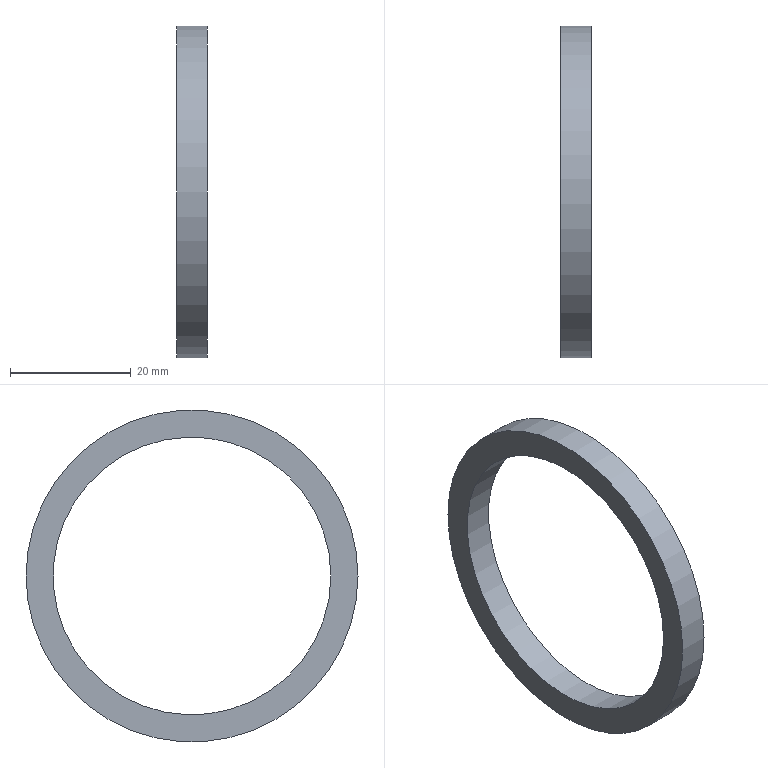Component | NX | XIAOTIAOZHENGHUAN_3 | 1 solid | 4 faces | box 5 x 55 x 55 mm | volume 3570 mm3 | cylinder 2 | plane 2 | commonest cylinder face diameters 55 x1 46 x1
STEP:
#1=CARTESIAN_POINT('',(0.,0.,0.));
#2=DIRECTION('',(0.,0.,1.));
#3=DIRECTION('',(1.,0.,0.));
#4=AXIS2_PLACEMENT_3D('',#1,#2,#3);
#5=CARTESIAN_POINT('',(-101.,-27.5,-88.));
#6=VERTEX_POINT('',#5);
#7=CARTESIAN_POINT('',(-101.,-0.,-88.));
#8=DIRECTION('',(-1.,0.,0.));
#9=DIRECTION('',(0.,-1.,0.));
#10=AXIS2_PLACEMENT_3D('',#7,#8,#9);
#11=CIRCLE('',#10,27.5);
#12=CARTESIAN_POINT('',(-101.,-0.,-88.));
#13=DIRECTION('',(1.,0.,0.));
#14=DIRECTION('',(0.,0.,1.));
#15=AXIS2_PLACEMENT_3D('',#12,#13,#14);
#16=CYLINDRICAL_SURFACE('',#15,27.5);
#17=CARTESIAN_POINT('',(7.854,0.));
#18=DIRECTION('',(-1.,0.));
#19=VECTOR('',#18,1.);
#20=LINE('',#17,#19);
#21=(GEOMETRIC_REPRESENTATION_CONTEXT(2)PARAMETRIC_REPRESENTATION_CONTEXT()REPRESENTATION_CONTEXT('',''));
#22=DEFINITIONAL_REPRESENTATION('',(#20),#21);
#23=PCURVE('',#16,#22);
#24=CARTESIAN_POINT('',(-101.,-0.,-88.));
#25=DIRECTION('',(-1.,0.,0.));
#26=DIRECTION('',(0.,0.,-1.));
#27=AXIS2_PLACEMENT_3D('',#24,#25,#26);
#28=PLANE('',#27);
#29=CARTESIAN_POINT('',(0.,0.));
#30=DIRECTION('',(0.,1.));
#31=AXIS2_PLACEMENT_2D('',#29,#30);
#32=CIRCLE('',#31,27.5);
#33=(GEOMETRIC_REPRESENTATION_CONTEXT(2)PARAMETRIC_REPRESENTATION_CONTEXT()REPRESENTATION_CONTEXT('',''));
#34=DEFINITIONAL_REPRESENTATION('',(#32),#33);
#35=PCURVE('',#28,#34);
#36=SURFACE_CURVE('',#11,(#23,#35),.PCURVE_S1.);
#37=EDGE_CURVE('',#6,#6,#36,.T.);
#38=ORIENTED_EDGE('',*,*,#37,.F.);
#39=CARTESIAN_POINT('',(-96.,-27.5,-88.));
#40=VERTEX_POINT('',#39);
#41=CARTESIAN_POINT('',(-101.,-27.5,-88.));
#42=CARTESIAN_POINT('',(-96.,-27.5,-88.));
#43=B_SPLINE_CURVE_WITH_KNOTS('',1,(#41,#42),.UNSPECIFIED.,.F.,.F.,(2,2),(0.,5.),.PIECEWISE_BEZIER_KNOTS.);
#44=CARTESIAN_POINT('',(7.854,0.));
#45=DIRECTION('',(0.,1.));
#46=VECTOR('',#45,1.);
#47=LINE('',#44,#46);
#48=(GEOMETRIC_REPRESENTATION_CONTEXT(2)PARAMETRIC_REPRESENTATION_CONTEXT()REPRESENTATION_CONTEXT('',''));
#49=DEFINITIONAL_REPRESENTATION('',(#47),#48);
#50=PCURVE('',#16,#49);
#51=CARTESIAN_POINT('',(1.571,0.));
#52=DIRECTION('',(0.,1.));
#53=VECTOR('',#52,1.);
#54=LINE('',#51,#53);
#55=(GEOMETRIC_REPRESENTATION_CONTEXT(2)PARAMETRIC_REPRESENTATION_CONTEXT()REPRESENTATION_CONTEXT('',''));
#56=DEFINITIONAL_REPRESENTATION('',(#54),#55);
#57=PCURVE('',#16,#56);
#58=SEAM_CURVE('',#43,(#50,#57),.PCURVE_S1.);
#59=EDGE_CURVE('',#6,#40,#58,.T.);
#60=ORIENTED_EDGE('',*,*,#59,.T.);
#61=CARTESIAN_POINT('',(-96.,-0.,-88.));
#62=DIRECTION('',(-1.,0.,0.));
#63=DIRECTION('',(0.,-1.,0.));
#64=AXIS2_PLACEMENT_3D('',#61,#62,#63);
#65=CIRCLE('',#64,27.5);
#66=CARTESIAN_POINT('',(7.854,5.));
#67=DIRECTION('',(-1.,0.));
#68=VECTOR('',#67,1.);
#69=LINE('',#66,#68);
#70=(GEOMETRIC_REPRESENTATION_CONTEXT(2)PARAMETRIC_REPRESENTATION_CONTEXT()REPRESENTATION_CONTEXT('',''));
#71=DEFINITIONAL_REPRESENTATION('',(#69),#70);
#72=PCURVE('',#16,#71);
#73=CARTESIAN_POINT('',(-96.,-0.,-88.));
#74=DIRECTION('',(-1.,0.,0.));
#75=DIRECTION('',(0.,0.,-1.));
#76=AXIS2_PLACEMENT_3D('',#73,#74,#75);
#77=PLANE('',#76);
#78=CARTESIAN_POINT('',(0.,0.));
#79=DIRECTION('',(0.,1.));
#80=AXIS2_PLACEMENT_2D('',#78,#79);
#81=CIRCLE('',#80,27.5);
#82=(GEOMETRIC_REPRESENTATION_CONTEXT(2)PARAMETRIC_REPRESENTATION_CONTEXT()REPRESENTATION_CONTEXT('',''));
#83=DEFINITIONAL_REPRESENTATION('',(#81),#82);
#84=PCURVE('',#77,#83);
#85=SURFACE_CURVE('',#65,(#72,#84),.PCURVE_S1.);
#86=EDGE_CURVE('',#40,#40,#85,.T.);
#87=ORIENTED_EDGE('',*,*,#86,.T.);
#88=ORIENTED_EDGE('',*,*,#59,.F.);
#89=EDGE_LOOP('',(#38,#60,#87,#88));
#90=FACE_BOUND('',#89,.T.);
#91=ADVANCED_FACE('',(#90),#16,.T.);
#92=CARTESIAN_POINT('',(-101.,-23.,-88.));
#93=VERTEX_POINT('',#92);
#94=CARTESIAN_POINT('',(-101.,-0.,-88.));
#95=DIRECTION('',(-1.,0.,0.));
#96=DIRECTION('',(0.,-1.,0.));
#97=AXIS2_PLACEMENT_3D('',#94,#95,#96);
#98=CIRCLE('',#97,23.);
#99=CARTESIAN_POINT('',(-101.,-0.,-88.));
#100=DIRECTION('',(1.,0.,0.));
#101=DIRECTION('',(0.,0.,1.));
#102=AXIS2_PLACEMENT_3D('',#99,#100,#101);
#103=CYLINDRICAL_SURFACE('',#102,23.);
#104=CARTESIAN_POINT('',(7.854,0.));
#105=DIRECTION('',(-1.,0.));
#106=VECTOR('',#105,1.);
#107=LINE('',#104,#106);
#108=(GEOMETRIC_REPRESENTATION_CONTEXT(2)PARAMETRIC_REPRESENTATION_CONTEXT()REPRESENTATION_CONTEXT('',''));
#109=DEFINITIONAL_REPRESENTATION('',(#107),#108);
#110=PCURVE('',#103,#109);
#111=CARTESIAN_POINT('',(0.,0.));
#112=DIRECTION('',(0.,1.));
#113=AXIS2_PLACEMENT_2D('',#111,#112);
#114=CIRCLE('',#113,23.);
#115=(GEOMETRIC_REPRESENTATION_CONTEXT(2)PARAMETRIC_REPRESENTATION_CONTEXT()REPRESENTATION_CONTEXT('',''));
#116=DEFINITIONAL_REPRESENTATION('',(#114),#115);
#117=PCURVE('',#28,#116);
#118=SURFACE_CURVE('',#98,(#110,#117),.PCURVE_S1.);
#119=EDGE_CURVE('',#93,#93,#118,.T.);
#120=ORIENTED_EDGE('',*,*,#119,.F.);
#121=CARTESIAN_POINT('',(-96.,-23.,-88.));
#122=VERTEX_POINT('',#121);
#123=CARTESIAN_POINT('',(-101.,-23.,-88.));
#124=CARTESIAN_POINT('',(-96.,-23.,-88.));
#125=B_SPLINE_CURVE_WITH_KNOTS('',1,(#123,#124),.UNSPECIFIED.,.F.,.F.,(2,2),(0.,5.),.PIECEWISE_BEZIER_KNOTS.);
#126=CARTESIAN_POINT('',(7.854,0.));
#127=DIRECTION('',(0.,1.));
#128=VECTOR('',#127,1.);
#129=LINE('',#126,#128);
#130=(GEOMETRIC_REPRESENTATION_CONTEXT(2)PARAMETRIC_REPRESENTATION_CONTEXT()REPRESENTATION_CONTEXT('',''));
#131=DEFINITIONAL_REPRESENTATION('',(#129),#130);
#132=PCURVE('',#103,#131);
#133=CARTESIAN_POINT('',(1.571,0.));
#134=DIRECTION('',(0.,1.));
#135=VECTOR('',#134,1.);
#136=LINE('',#133,#135);
#137=(GEOMETRIC_REPRESENTATION_CONTEXT(2)PARAMETRIC_REPRESENTATION_CONTEXT()REPRESENTATION_CONTEXT('',''));
#138=DEFINITIONAL_REPRESENTATION('',(#136),#137);
#139=PCURVE('',#103,#138);
#140=SEAM_CURVE('',#125,(#132,#139),.PCURVE_S1.);
#141=EDGE_CURVE('',#93,#122,#140,.T.);
#142=ORIENTED_EDGE('',*,*,#141,.T.);
#143=CARTESIAN_POINT('',(-96.,-0.,-88.));
#144=DIRECTION('',(-1.,0.,0.));
#145=DIRECTION('',(0.,-1.,0.));
#146=AXIS2_PLACEMENT_3D('',#143,#144,#145);
#147=CIRCLE('',#146,23.);
#148=CARTESIAN_POINT('',(7.854,5.));
#149=DIRECTION('',(-1.,0.));
#150=VECTOR('',#149,1.);
#151=LINE('',#148,#150);
#152=(GEOMETRIC_REPRESENTATION_CONTEXT(2)PARAMETRIC_REPRESENTATION_CONTEXT()REPRESENTATION_CONTEXT('',''));
#153=DEFINITIONAL_REPRESENTATION('',(#151),#152);
#154=PCURVE('',#103,#153);
#155=CARTESIAN_POINT('',(0.,0.));
#156=DIRECTION('',(0.,1.));
#157=AXIS2_PLACEMENT_2D('',#155,#156);
#158=CIRCLE('',#157,23.);
#159=(GEOMETRIC_REPRESENTATION_CONTEXT(2)PARAMETRIC_REPRESENTATION_CONTEXT()REPRESENTATION_CONTEXT('',''));
#160=DEFINITIONAL_REPRESENTATION('',(#158),#159);
#161=PCURVE('',#77,#160);
#162=SURFACE_CURVE('',#147,(#154,#161),.PCURVE_S1.);
#163=EDGE_CURVE('',#122,#122,#162,.T.);
#164=ORIENTED_EDGE('',*,*,#163,.T.);
#165=ORIENTED_EDGE('',*,*,#141,.F.);
#166=EDGE_LOOP('',(#120,#142,#164,#165));
#167=FACE_BOUND('',#166,.F.);
#168=ADVANCED_FACE('',(#167),#103,.F.);
#169=ORIENTED_EDGE('',*,*,#37,.T.);
#170=EDGE_LOOP('',(#169));
#171=FACE_BOUND('',#170,.T.);
#172=ORIENTED_EDGE('',*,*,#119,.F.);
#173=EDGE_LOOP('',(#172));
#174=FACE_BOUND('',#173,.T.);
#175=ADVANCED_FACE('',(#171,#174),#28,.T.);
#176=ORIENTED_EDGE('',*,*,#86,.F.);
#177=EDGE_LOOP('',(#176));
#178=FACE_BOUND('',#177,.T.);
#179=ORIENTED_EDGE('',*,*,#163,.T.);
#180=EDGE_LOOP('',(#179));
#181=FACE_BOUND('',#180,.T.);
#182=ADVANCED_FACE('',(#178,#181),#77,.F.);
#183=CLOSED_SHELL('',(#91,#168,#175,#182));
#184=MANIFOLD_SOLID_BREP('',#183);
#185=(LENGTH_UNIT()NAMED_UNIT(*)SI_UNIT(.MILLI.,.METRE.));
#186=UNCERTAINTY_MEASURE_WITH_UNIT(LENGTH_MEASURE(0.00001),#185,'','');
#187=(NAMED_UNIT(*)PLANE_ANGLE_UNIT()SI_UNIT($,.RADIAN.));
#188=(NAMED_UNIT(*)SI_UNIT($,.STERADIAN.)SOLID_ANGLE_UNIT());
#189=(GEOMETRIC_REPRESENTATION_CONTEXT(3)GLOBAL_UNCERTAINTY_ASSIGNED_CONTEXT((#186))GLOBAL_UNIT_ASSIGNED_CONTEXT((#185,#187,#188))REPRESENTATION_CONTEXT('',''));
#190=ADVANCED_BREP_SHAPE_REPRESENTATION('',(#4,#184),#189);